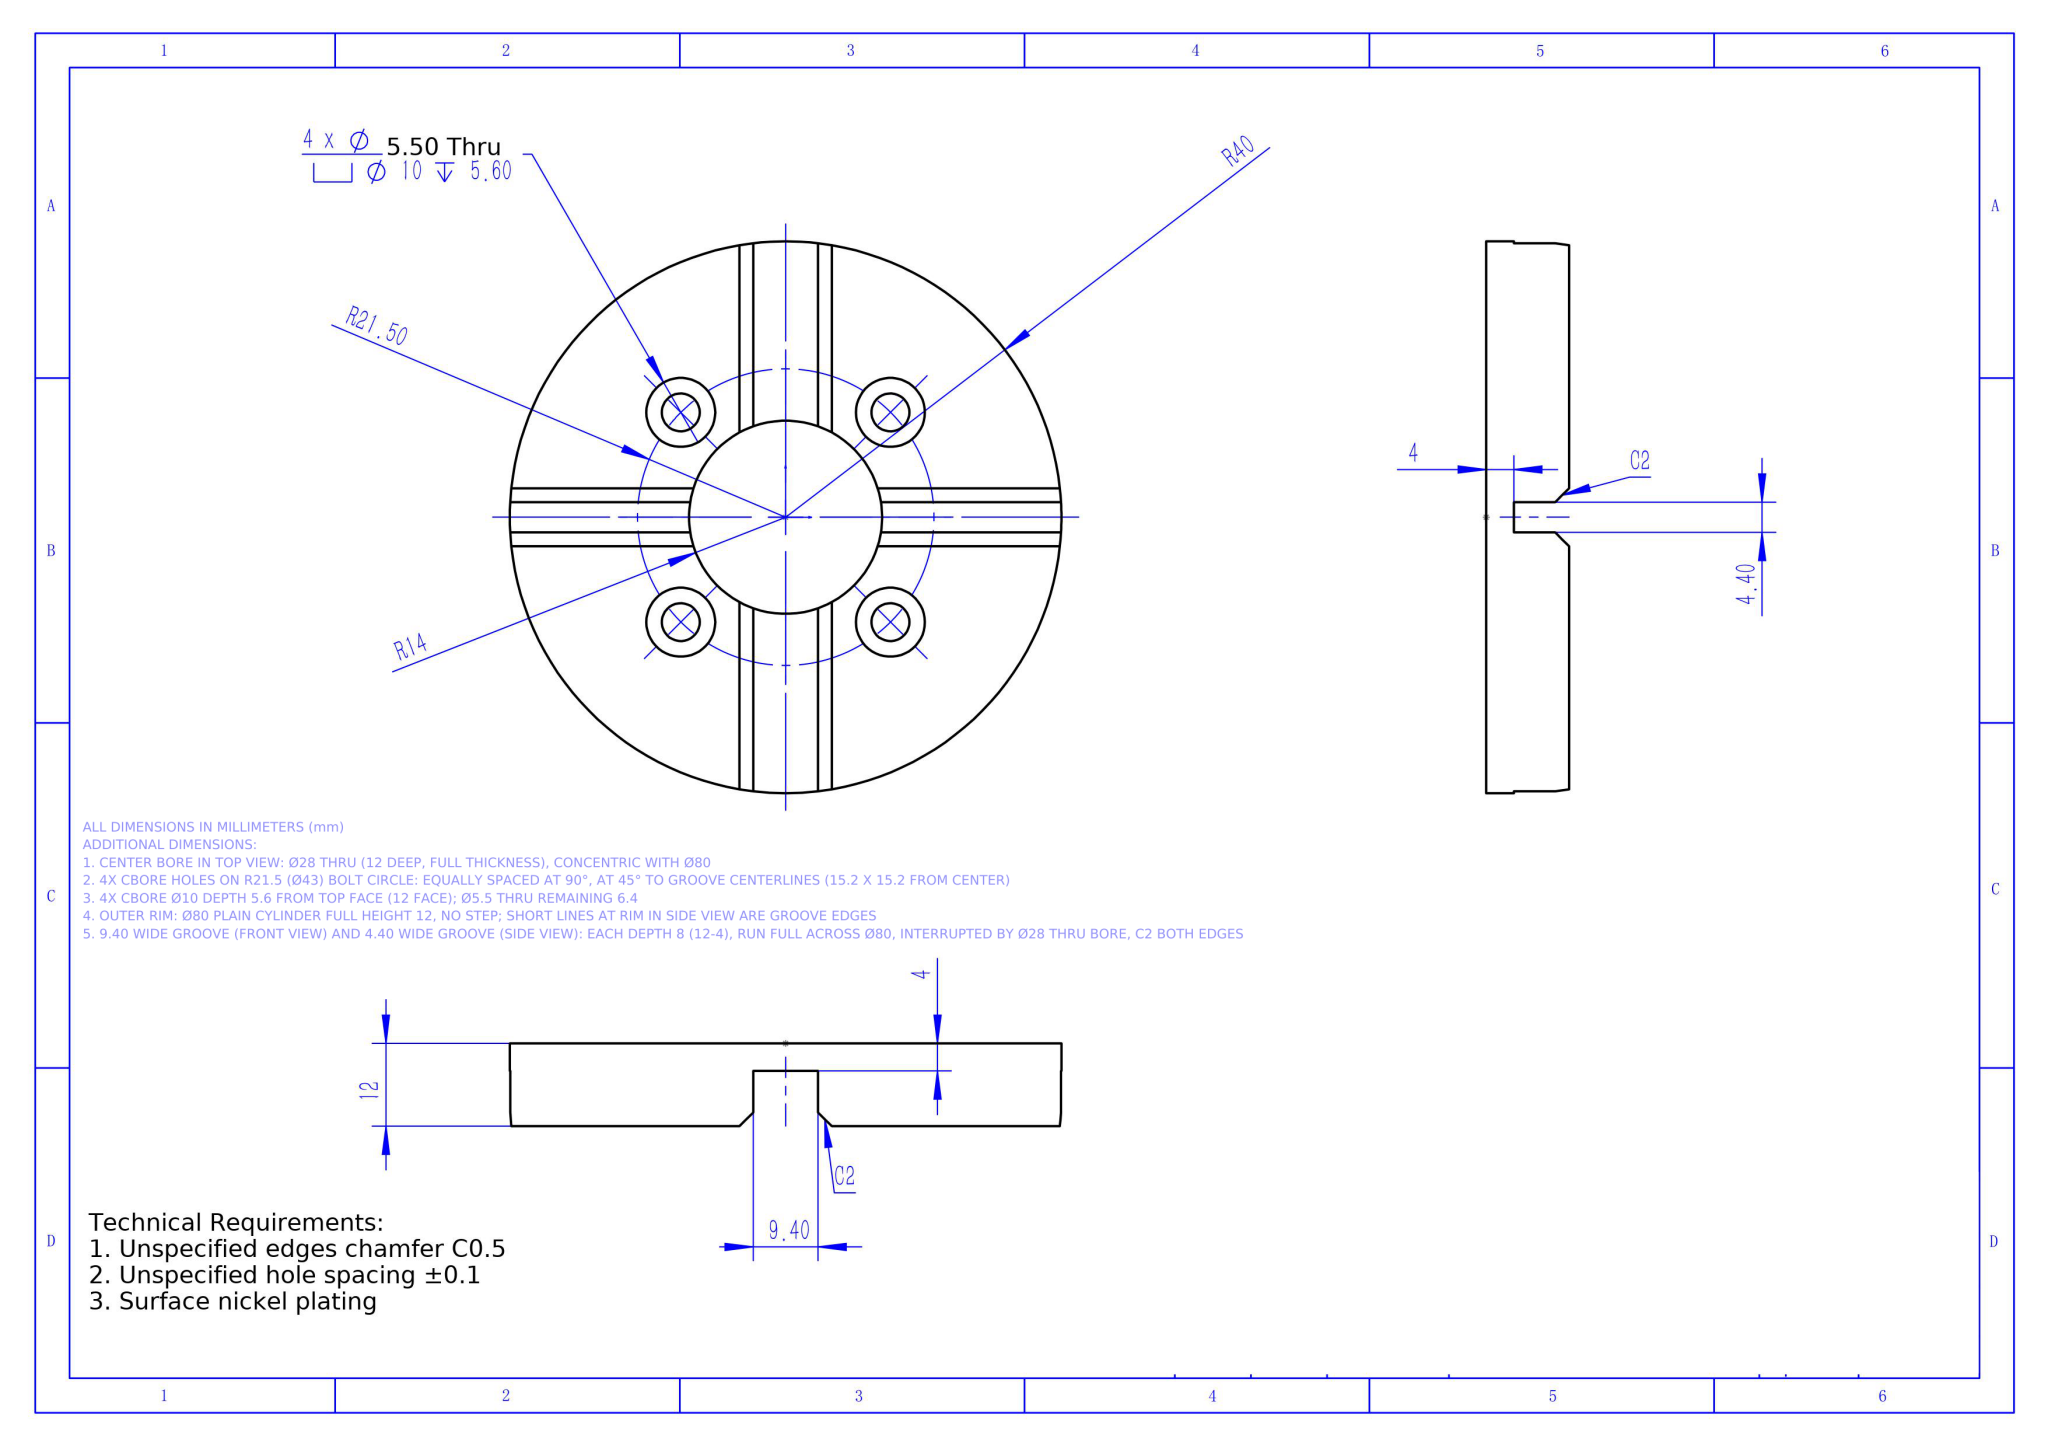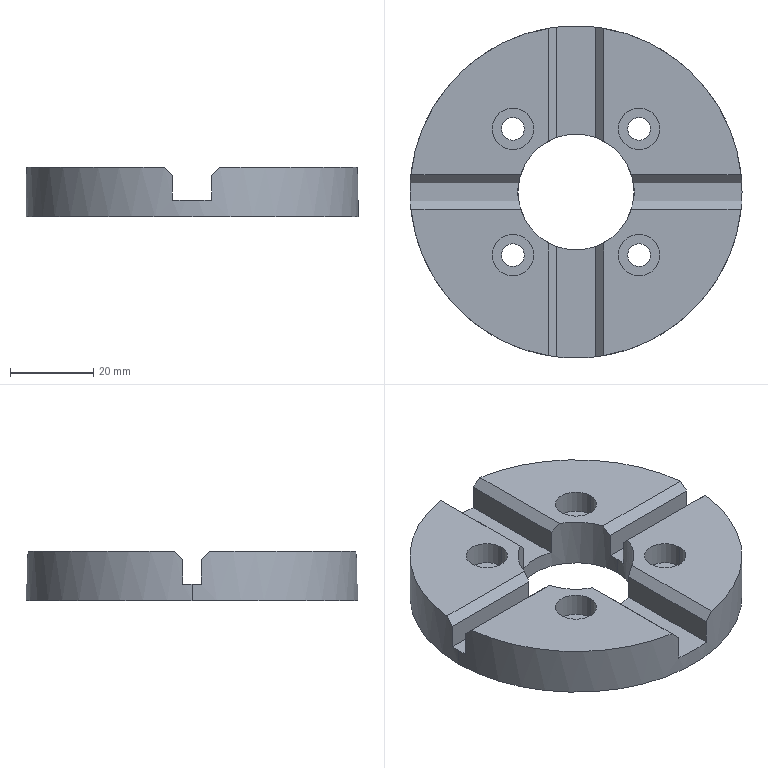Part | NX | mm | 1 solid | 49 faces | box 80 x 80 x 12 mm | volume 44369 mm3 | plane 29 | cylinder 20 | commonest cylinder face diameters 10 x8 5.5 x8 28 x2 80 x2